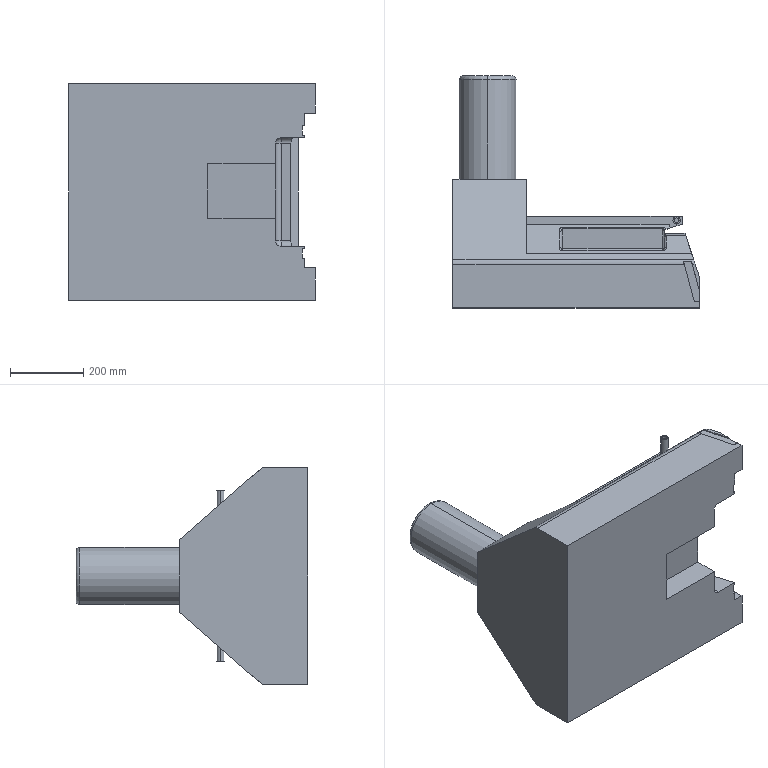Component | SolidWorks | RehabilitationChair-18-15-1 | 3 solids | 155 faces | volume 82002158 mm3 | plane 84 | cylinder 55 | spline 8 | sphere 6 | torus 2 | commonest cylinder face diameters 10 x18 13 x8 30 x5 20.089 x4 40 x4 20.116 x4 134.252 x2 155.793 x2